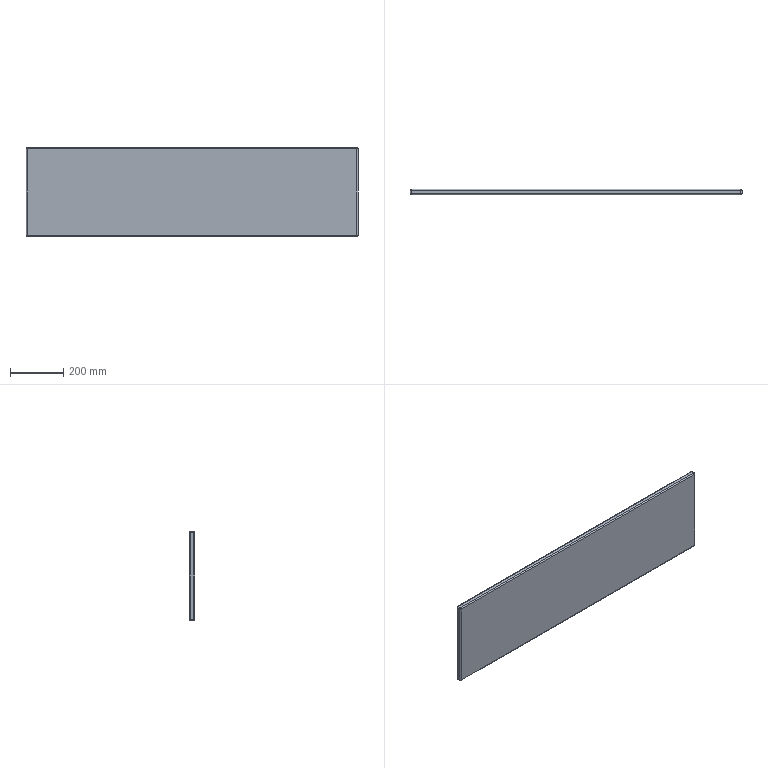Component | SolidWorks | AX00-100.1.1-1_25.1.1-1 | 1 solid | 26 faces | box 1243 x 20 x 333 mm | volume 8256545 mm3 | cylinder 12 | sphere 8 | plane 6 | commonest cylinder face diameters 8 x12
build123d program:
from build123d import *

# Parameters (mm, degrees)
SKETCH1_W           = 1243
SKETCH1_H           = 333
BOSS_EXTRUDE1_DEPTH = 10
FILLET1_R           = 4
FILLET2_R           = 4


with BuildPart() as part:
    # Sketch1 → Boss-Extrude1 (new, symmetric)
    with BuildSketch(Plane.XY):
        Rectangle(SKETCH1_W, SKETCH1_H)
    extrude(amount=BOSS_EXTRUDE1_DEPTH, both=True)

    # Fillet1
    fillet1_edges = [part.edges().sort_by_distance(p)[0] for p in [
        (621.5, -166.5, 0),
        (-621.5, -166.5, 0),
        (-621.5, 166.5, 0),
        (621.5, 166.5, 0),
    ]]
    fillet(fillet1_edges, radius=FILLET1_R)

    # Fillet2
    fillet2_edges = [part.edges().sort_by_distance(p)[0] for p in [
        (0, -166.5, -10),
        (0, -166.5, 10),
        (621.5, 0, -10),
        (-621.5, 0, -10),
        (0, 166.5, -10),
        (620.328, 165.328, -10),
        (620.328, -165.328, -10),
        (-620.328, 165.328, -10),
        (-620.328, -165.328, -10),
        (-621.5, 0, 10),
        (621.5, 0, 10),
        (0, 166.5, 10),
        (620.328, 165.328, 10),
        (620.328, -165.328, 10),
        (-620.328, 165.328, 10),
        (-620.328, -165.328, 10),
    ]]
    fillet(fillet2_edges, radius=FILLET2_R)


solid = part.part

# Placed as in the assembly
solid = solid.moved(Location((-38.869, -376.636, -5), (90, 0, 0)))